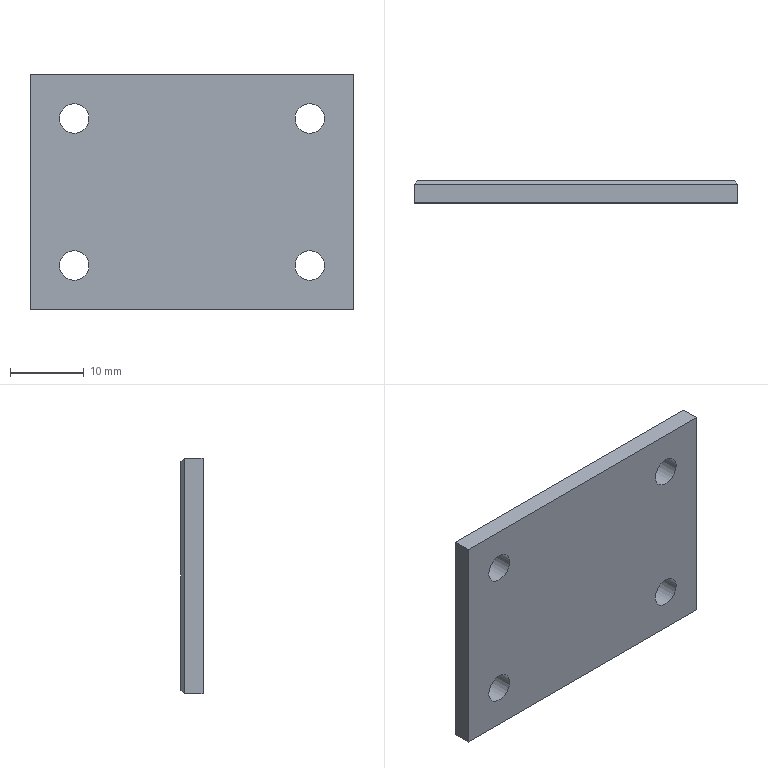Component | NX | END_CAP | 1 solid | 14 faces | box 44 x 3 x 32 mm | volume 4054 mm3 | plane 10 | cylinder 4 | commonest cylinder face diameters 4 x4
STEP:
#1=CARTESIAN_POINT('',(0.,0.,0.));
#2=DIRECTION('',(0.,0.,1.));
#3=DIRECTION('',(1.,0.,0.));
#4=AXIS2_PLACEMENT_3D('',#1,#2,#3);
#5=CARTESIAN_POINT('',(412.5,-54.,127.));
#6=VERTEX_POINT('',#5);
#7=CARTESIAN_POINT('',(412.5,-56.5,127.));
#8=VERTEX_POINT('',#7);
#9=CARTESIAN_POINT('',(412.5,-53.5,127.));
#10=DIRECTION('',(0.,-1.,0.));
#11=VECTOR('',#10,1.);
#12=LINE('',#9,#11);
#13=CARTESIAN_POINT('',(412.5,-53.5,127.));
#14=DIRECTION('',(0.,0.,1.));
#15=DIRECTION('',(0.,-1.,0.));
#16=AXIS2_PLACEMENT_3D('',#13,#14,#15);
#17=PLANE('',#16);
#18=CARTESIAN_POINT('',(0.,0.));
#19=DIRECTION('',(1.,0.));
#20=VECTOR('',#19,1.);
#21=LINE('',#18,#20);
#22=(GEOMETRIC_REPRESENTATION_CONTEXT(2)PARAMETRIC_REPRESENTATION_CONTEXT()REPRESENTATION_CONTEXT('',''));
#23=DEFINITIONAL_REPRESENTATION('',(#21),#22);
#24=PCURVE('',#17,#23);
#25=CARTESIAN_POINT('',(412.5,-53.5,95.));
#26=DIRECTION('',(1.,0.,0.));
#27=DIRECTION('',(0.,-1.,0.));
#28=AXIS2_PLACEMENT_3D('',#25,#26,#27);
#29=PLANE('',#28);
#30=CARTESIAN_POINT('',(0.,-32.));
#31=DIRECTION('',(1.,0.));
#32=VECTOR('',#31,1.);
#33=LINE('',#30,#32);
#34=(GEOMETRIC_REPRESENTATION_CONTEXT(2)PARAMETRIC_REPRESENTATION_CONTEXT()REPRESENTATION_CONTEXT('',''));
#35=DEFINITIONAL_REPRESENTATION('',(#33),#34);
#36=PCURVE('',#29,#35);
#37=SURFACE_CURVE('',#12,(#24,#36),.PCURVE_S1.);
#38=EDGE_CURVE('',#6,#8,#37,.T.);
#39=ORIENTED_EDGE('',*,*,#38,.F.);
#40=CARTESIAN_POINT('',(368.5,-54.,127.));
#41=VERTEX_POINT('',#40);
#42=CARTESIAN_POINT('',(412.5,-54.,127.));
#43=DIRECTION('',(-1.,0.,0.));
#44=VECTOR('',#43,1.);
#45=LINE('',#42,#44);
#46=CARTESIAN_POINT('',(0.5,0.));
#47=DIRECTION('',(0.,-1.));
#48=VECTOR('',#47,1.);
#49=LINE('',#46,#48);
#50=(GEOMETRIC_REPRESENTATION_CONTEXT(2)PARAMETRIC_REPRESENTATION_CONTEXT()REPRESENTATION_CONTEXT('',''));
#51=DEFINITIONAL_REPRESENTATION('',(#49),#50);
#52=PCURVE('',#17,#51);
#53=CARTESIAN_POINT('',(412.5,-54.,127.));
#54=DIRECTION('',(0.,-0.7071,-0.7071));
#55=DIRECTION('',(-1.,0.,0.));
#56=AXIS2_PLACEMENT_3D('',#53,#54,#55);
#57=PLANE('',#56);
#58=CARTESIAN_POINT('',(0.,0.));
#59=DIRECTION('',(1.,0.));
#60=VECTOR('',#59,1.);
#61=LINE('',#58,#60);
#62=(GEOMETRIC_REPRESENTATION_CONTEXT(2)PARAMETRIC_REPRESENTATION_CONTEXT()REPRESENTATION_CONTEXT('',''));
#63=DEFINITIONAL_REPRESENTATION('',(#61),#62);
#64=PCURVE('',#57,#63);
#65=SURFACE_CURVE('',#45,(#52,#64),.PCURVE_S1.);
#66=EDGE_CURVE('',#6,#41,#65,.T.);
#67=ORIENTED_EDGE('',*,*,#66,.T.);
#68=CARTESIAN_POINT('',(368.5,-56.5,127.));
#69=VERTEX_POINT('',#68);
#70=CARTESIAN_POINT('',(368.5,-53.5,127.));
#71=DIRECTION('',(0.,-1.,0.));
#72=VECTOR('',#71,1.);
#73=LINE('',#70,#72);
#74=CARTESIAN_POINT('',(0.,-44.));
#75=DIRECTION('',(1.,0.));
#76=VECTOR('',#75,1.);
#77=LINE('',#74,#76);
#78=(GEOMETRIC_REPRESENTATION_CONTEXT(2)PARAMETRIC_REPRESENTATION_CONTEXT()REPRESENTATION_CONTEXT('',''));
#79=DEFINITIONAL_REPRESENTATION('',(#77),#78);
#80=PCURVE('',#17,#79);
#81=CARTESIAN_POINT('',(368.5,-53.5,127.));
#82=DIRECTION('',(-1.,0.,0.));
#83=DIRECTION('',(0.,1.,0.));
#84=AXIS2_PLACEMENT_3D('',#81,#82,#83);
#85=PLANE('',#84);
#86=CARTESIAN_POINT('',(0.,0.));
#87=DIRECTION('',(-1.,0.));
#88=VECTOR('',#87,1.);
#89=LINE('',#86,#88);
#90=(GEOMETRIC_REPRESENTATION_CONTEXT(2)PARAMETRIC_REPRESENTATION_CONTEXT()REPRESENTATION_CONTEXT('',''));
#91=DEFINITIONAL_REPRESENTATION('',(#89),#90);
#92=PCURVE('',#85,#91);
#93=SURFACE_CURVE('',#73,(#80,#92),.PCURVE_S1.);
#94=EDGE_CURVE('',#41,#69,#93,.T.);
#95=ORIENTED_EDGE('',*,*,#94,.T.);
#96=CARTESIAN_POINT('',(412.5,-56.5,127.));
#97=DIRECTION('',(-1.,0.,0.));
#98=VECTOR('',#97,1.);
#99=LINE('',#96,#98);
#100=CARTESIAN_POINT('',(3.,0.));
#101=DIRECTION('',(0.,-1.));
#102=VECTOR('',#101,1.);
#103=LINE('',#100,#102);
#104=(GEOMETRIC_REPRESENTATION_CONTEXT(2)PARAMETRIC_REPRESENTATION_CONTEXT()REPRESENTATION_CONTEXT('',''));
#105=DEFINITIONAL_REPRESENTATION('',(#103),#104);
#106=PCURVE('',#17,#105);
#107=CARTESIAN_POINT('',(406.5,-56.5,101.));
#108=DIRECTION('',(0.,1.,0.));
#109=DIRECTION('',(1.,0.,0.));
#110=AXIS2_PLACEMENT_3D('',#107,#108,#109);
#111=PLANE('',#110);
#112=CARTESIAN_POINT('',(6.,-26.));
#113=DIRECTION('',(-1.,0.));
#114=VECTOR('',#113,1.);
#115=LINE('',#112,#114);
#116=(GEOMETRIC_REPRESENTATION_CONTEXT(2)PARAMETRIC_REPRESENTATION_CONTEXT()REPRESENTATION_CONTEXT('',''));
#117=DEFINITIONAL_REPRESENTATION('',(#115),#116);
#118=PCURVE('',#111,#117);
#119=SURFACE_CURVE('',#99,(#106,#118),.PCURVE_S1.);
#120=EDGE_CURVE('',#8,#69,#119,.T.);
#121=ORIENTED_EDGE('',*,*,#120,.F.);
#122=EDGE_LOOP('',(#39,#67,#95,#121));
#123=FACE_BOUND('',#122,.T.);
#124=ADVANCED_FACE('',(#123),#17,.T.);
#125=ORIENTED_EDGE('',*,*,#94,.F.);
#126=CARTESIAN_POINT('',(368.5,-54.,95.));
#127=VERTEX_POINT('',#126);
#128=CARTESIAN_POINT('',(368.5,-54.,127.));
#129=DIRECTION('',(0.,0.,-1.));
#130=VECTOR('',#129,1.);
#131=LINE('',#128,#130);
#132=CARTESIAN_POINT('',(-0.5,0.));
#133=DIRECTION('',(0.,1.));
#134=VECTOR('',#133,1.);
#135=LINE('',#132,#134);
#136=(GEOMETRIC_REPRESENTATION_CONTEXT(2)PARAMETRIC_REPRESENTATION_CONTEXT()REPRESENTATION_CONTEXT('',''));
#137=DEFINITIONAL_REPRESENTATION('',(#135),#136);
#138=PCURVE('',#85,#137);
#139=CARTESIAN_POINT('',(368.5,-54.,127.));
#140=DIRECTION('',(0.7071,-0.7071,0.));
#141=DIRECTION('',(0.,0.,-1.));
#142=AXIS2_PLACEMENT_3D('',#139,#140,#141);
#143=PLANE('',#142);
#144=CARTESIAN_POINT('',(0.,0.));
#145=DIRECTION('',(1.,0.));
#146=VECTOR('',#145,1.);
#147=LINE('',#144,#146);
#148=(GEOMETRIC_REPRESENTATION_CONTEXT(2)PARAMETRIC_REPRESENTATION_CONTEXT()REPRESENTATION_CONTEXT('',''));
#149=DEFINITIONAL_REPRESENTATION('',(#147),#148);
#150=PCURVE('',#143,#149);
#151=SURFACE_CURVE('',#131,(#138,#150),.PCURVE_S1.);
#152=EDGE_CURVE('',#41,#127,#151,.T.);
#153=ORIENTED_EDGE('',*,*,#152,.T.);
#154=CARTESIAN_POINT('',(368.5,-56.5,95.));
#155=VERTEX_POINT('',#154);
#156=CARTESIAN_POINT('',(368.5,-53.5,95.));
#157=DIRECTION('',(0.,-1.,0.));
#158=VECTOR('',#157,1.);
#159=LINE('',#156,#158);
#160=CARTESIAN_POINT('',(0.,32.));
#161=DIRECTION('',(-1.,0.));
#162=VECTOR('',#161,1.);
#163=LINE('',#160,#162);
#164=(GEOMETRIC_REPRESENTATION_CONTEXT(2)PARAMETRIC_REPRESENTATION_CONTEXT()REPRESENTATION_CONTEXT('',''));
#165=DEFINITIONAL_REPRESENTATION('',(#163),#164);
#166=PCURVE('',#85,#165);
#167=CARTESIAN_POINT('',(368.5,-53.5,95.));
#168=DIRECTION('',(0.,0.,-1.));
#169=DIRECTION('',(0.,1.,0.));
#170=AXIS2_PLACEMENT_3D('',#167,#168,#169);
#171=PLANE('',#170);
#172=CARTESIAN_POINT('',(0.,0.));
#173=DIRECTION('',(-1.,0.));
#174=VECTOR('',#173,1.);
#175=LINE('',#172,#174);
#176=(GEOMETRIC_REPRESENTATION_CONTEXT(2)PARAMETRIC_REPRESENTATION_CONTEXT()REPRESENTATION_CONTEXT('',''));
#177=DEFINITIONAL_REPRESENTATION('',(#175),#176);
#178=PCURVE('',#171,#177);
#179=SURFACE_CURVE('',#159,(#166,#178),.PCURVE_S1.);
#180=EDGE_CURVE('',#127,#155,#179,.T.);
#181=ORIENTED_EDGE('',*,*,#180,.T.);
#182=CARTESIAN_POINT('',(368.5,-56.5,127.));
#183=DIRECTION('',(0.,0.,-1.));
#184=VECTOR('',#183,1.);
#185=LINE('',#182,#184);
#186=CARTESIAN_POINT('',(-3.,0.));
#187=DIRECTION('',(0.,1.));
#188=VECTOR('',#187,1.);
#189=LINE('',#186,#188);
#190=(GEOMETRIC_REPRESENTATION_CONTEXT(2)PARAMETRIC_REPRESENTATION_CONTEXT()REPRESENTATION_CONTEXT('',''));
#191=DEFINITIONAL_REPRESENTATION('',(#189),#190);
#192=PCURVE('',#85,#191);
#193=CARTESIAN_POINT('',(-38.,-26.));
#194=DIRECTION('',(0.,1.));
#195=VECTOR('',#194,1.);
#196=LINE('',#193,#195);
#197=(GEOMETRIC_REPRESENTATION_CONTEXT(2)PARAMETRIC_REPRESENTATION_CONTEXT()REPRESENTATION_CONTEXT('',''));
#198=DEFINITIONAL_REPRESENTATION('',(#196),#197);
#199=PCURVE('',#111,#198);
#200=SURFACE_CURVE('',#185,(#192,#199),.PCURVE_S1.);
#201=EDGE_CURVE('',#69,#155,#200,.T.);
#202=ORIENTED_EDGE('',*,*,#201,.F.);
#203=EDGE_LOOP('',(#125,#153,#181,#202));
#204=FACE_BOUND('',#203,.T.);
#205=ADVANCED_FACE('',(#204),#85,.T.);
#206=ORIENTED_EDGE('',*,*,#180,.F.);
#207=CARTESIAN_POINT('',(412.5,-54.,95.));
#208=VERTEX_POINT('',#207);
#209=CARTESIAN_POINT('',(368.5,-54.,95.));
#210=DIRECTION('',(1.,0.,0.));
#211=VECTOR('',#210,1.);
#212=LINE('',#209,#211);
#213=CARTESIAN_POINT('',(-0.5,0.));
#214=DIRECTION('',(0.,1.));
#215=VECTOR('',#214,1.);
#216=LINE('',#213,#215);
#217=(GEOMETRIC_REPRESENTATION_CONTEXT(2)PARAMETRIC_REPRESENTATION_CONTEXT()REPRESENTATION_CONTEXT('',''));
#218=DEFINITIONAL_REPRESENTATION('',(#216),#217);
#219=PCURVE('',#171,#218);
#220=CARTESIAN_POINT('',(368.5,-54.,95.));
#221=DIRECTION('',(0.,-0.7071,0.7071));
#222=DIRECTION('',(1.,0.,0.));
#223=AXIS2_PLACEMENT_3D('',#220,#221,#222);
#224=PLANE('',#223);
#225=CARTESIAN_POINT('',(0.,0.));
#226=DIRECTION('',(1.,0.));
#227=VECTOR('',#226,1.);
#228=LINE('',#225,#227);
#229=(GEOMETRIC_REPRESENTATION_CONTEXT(2)PARAMETRIC_REPRESENTATION_CONTEXT()REPRESENTATION_CONTEXT('',''));
#230=DEFINITIONAL_REPRESENTATION('',(#228),#229);
#231=PCURVE('',#224,#230);
#232=SURFACE_CURVE('',#212,(#219,#231),.PCURVE_S1.);
#233=EDGE_CURVE('',#127,#208,#232,.T.);
#234=ORIENTED_EDGE('',*,*,#233,.T.);
#235=CARTESIAN_POINT('',(412.5,-56.5,95.));
#236=VERTEX_POINT('',#235);
#237=CARTESIAN_POINT('',(412.5,-53.5,95.));
#238=DIRECTION('',(0.,-1.,0.));
#239=VECTOR('',#238,1.);
#240=LINE('',#237,#239);
#241=CARTESIAN_POINT('',(0.,44.));
#242=DIRECTION('',(-1.,0.));
#243=VECTOR('',#242,1.);
#244=LINE('',#241,#243);
#245=(GEOMETRIC_REPRESENTATION_CONTEXT(2)PARAMETRIC_REPRESENTATION_CONTEXT()REPRESENTATION_CONTEXT('',''));
#246=DEFINITIONAL_REPRESENTATION('',(#244),#245);
#247=PCURVE('',#171,#246);
#248=CARTESIAN_POINT('',(0.,0.));
#249=DIRECTION('',(1.,0.));
#250=VECTOR('',#249,1.);
#251=LINE('',#248,#250);
#252=(GEOMETRIC_REPRESENTATION_CONTEXT(2)PARAMETRIC_REPRESENTATION_CONTEXT()REPRESENTATION_CONTEXT('',''));
#253=DEFINITIONAL_REPRESENTATION('',(#251),#252);
#254=PCURVE('',#29,#253);
#255=SURFACE_CURVE('',#240,(#247,#254),.PCURVE_S1.);
#256=EDGE_CURVE('',#208,#236,#255,.T.);
#257=ORIENTED_EDGE('',*,*,#256,.T.);
#258=CARTESIAN_POINT('',(368.5,-56.5,95.));
#259=DIRECTION('',(1.,0.,0.));
#260=VECTOR('',#259,1.);
#261=LINE('',#258,#260);
#262=CARTESIAN_POINT('',(-3.,0.));
#263=DIRECTION('',(0.,1.));
#264=VECTOR('',#263,1.);
#265=LINE('',#262,#264);
#266=(GEOMETRIC_REPRESENTATION_CONTEXT(2)PARAMETRIC_REPRESENTATION_CONTEXT()REPRESENTATION_CONTEXT('',''));
#267=DEFINITIONAL_REPRESENTATION('',(#265),#266);
#268=PCURVE('',#171,#267);
#269=CARTESIAN_POINT('',(-38.,6.));
#270=DIRECTION('',(1.,0.));
#271=VECTOR('',#270,1.);
#272=LINE('',#269,#271);
#273=(GEOMETRIC_REPRESENTATION_CONTEXT(2)PARAMETRIC_REPRESENTATION_CONTEXT()REPRESENTATION_CONTEXT('',''));
#274=DEFINITIONAL_REPRESENTATION('',(#272),#273);
#275=PCURVE('',#111,#274);
#276=SURFACE_CURVE('',#261,(#268,#275),.PCURVE_S1.);
#277=EDGE_CURVE('',#155,#236,#276,.T.);
#278=ORIENTED_EDGE('',*,*,#277,.F.);
#279=EDGE_LOOP('',(#206,#234,#257,#278));
#280=FACE_BOUND('',#279,.T.);
#281=ADVANCED_FACE('',(#280),#171,.T.);
#282=CARTESIAN_POINT('',(376.5,-53.5,121.));
#283=VERTEX_POINT('',#282);
#284=CARTESIAN_POINT('',(374.5,-53.5,121.));
#285=DIRECTION('',(0.,1.,0.));
#286=DIRECTION('',(1.,0.,0.));
#287=AXIS2_PLACEMENT_3D('',#284,#285,#286);
#288=CIRCLE('',#287,2.);
#289=CARTESIAN_POINT('',(374.5,-53.5,121.));
#290=DIRECTION('',(0.,-1.,0.));
#291=DIRECTION('',(-1.,0.,0.));
#292=AXIS2_PLACEMENT_3D('',#289,#290,#291);
#293=CYLINDRICAL_SURFACE('',#292,2.);
#294=CARTESIAN_POINT('',(9.425,0.));
#295=DIRECTION('',(-1.,0.));
#296=VECTOR('',#295,1.);
#297=LINE('',#294,#296);
#298=(GEOMETRIC_REPRESENTATION_CONTEXT(2)PARAMETRIC_REPRESENTATION_CONTEXT()REPRESENTATION_CONTEXT('',''));
#299=DEFINITIONAL_REPRESENTATION('',(#297),#298);
#300=PCURVE('',#293,#299);
#301=CARTESIAN_POINT('',(406.5,-53.5,101.));
#302=DIRECTION('',(0.,1.,0.));
#303=DIRECTION('',(1.,0.,0.));
#304=AXIS2_PLACEMENT_3D('',#301,#302,#303);
#305=PLANE('',#304);
#306=CARTESIAN_POINT('',(-32.,-20.));
#307=DIRECTION('',(1.,0.));
#308=AXIS2_PLACEMENT_2D('',#306,#307);
#309=CIRCLE('',#308,2.);
#310=(GEOMETRIC_REPRESENTATION_CONTEXT(2)PARAMETRIC_REPRESENTATION_CONTEXT()REPRESENTATION_CONTEXT('',''));
#311=DEFINITIONAL_REPRESENTATION('',(#309),#310);
#312=PCURVE('',#305,#311);
#313=SURFACE_CURVE('',#288,(#300,#312),.PCURVE_S1.);
#314=EDGE_CURVE('',#283,#283,#313,.T.);
#315=ORIENTED_EDGE('',*,*,#314,.F.);
#316=CARTESIAN_POINT('',(376.5,-56.5,121.));
#317=VERTEX_POINT('',#316);
#318=CARTESIAN_POINT('',(376.5,-53.5,121.));
#319=CARTESIAN_POINT('',(376.5,-56.5,121.));
#320=B_SPLINE_CURVE_WITH_KNOTS('',1,(#318,#319),.UNSPECIFIED.,.F.,.F.,(2,2),(0.,3.),.PIECEWISE_BEZIER_KNOTS.);
#321=CARTESIAN_POINT('',(9.425,0.));
#322=DIRECTION('',(0.,1.));
#323=VECTOR('',#322,1.);
#324=LINE('',#321,#323);
#325=(GEOMETRIC_REPRESENTATION_CONTEXT(2)PARAMETRIC_REPRESENTATION_CONTEXT()REPRESENTATION_CONTEXT('',''));
#326=DEFINITIONAL_REPRESENTATION('',(#324),#325);
#327=PCURVE('',#293,#326);
#328=CARTESIAN_POINT('',(3.142,0.));
#329=DIRECTION('',(0.,1.));
#330=VECTOR('',#329,1.);
#331=LINE('',#328,#330);
#332=(GEOMETRIC_REPRESENTATION_CONTEXT(2)PARAMETRIC_REPRESENTATION_CONTEXT()REPRESENTATION_CONTEXT('',''));
#333=DEFINITIONAL_REPRESENTATION('',(#331),#332);
#334=PCURVE('',#293,#333);
#335=SEAM_CURVE('',#320,(#327,#334),.PCURVE_S1.);
#336=EDGE_CURVE('',#283,#317,#335,.T.);
#337=ORIENTED_EDGE('',*,*,#336,.T.);
#338=CARTESIAN_POINT('',(374.5,-56.5,121.));
#339=DIRECTION('',(0.,1.,0.));
#340=DIRECTION('',(1.,0.,0.));
#341=AXIS2_PLACEMENT_3D('',#338,#339,#340);
#342=CIRCLE('',#341,2.);
#343=CARTESIAN_POINT('',(9.425,3.));
#344=DIRECTION('',(-1.,0.));
#345=VECTOR('',#344,1.);
#346=LINE('',#343,#345);
#347=(GEOMETRIC_REPRESENTATION_CONTEXT(2)PARAMETRIC_REPRESENTATION_CONTEXT()REPRESENTATION_CONTEXT('',''));
#348=DEFINITIONAL_REPRESENTATION('',(#346),#347);
#349=PCURVE('',#293,#348);
#350=CARTESIAN_POINT('',(-32.,-20.));
#351=DIRECTION('',(1.,0.));
#352=AXIS2_PLACEMENT_2D('',#350,#351);
#353=CIRCLE('',#352,2.);
#354=(GEOMETRIC_REPRESENTATION_CONTEXT(2)PARAMETRIC_REPRESENTATION_CONTEXT()REPRESENTATION_CONTEXT('',''));
#355=DEFINITIONAL_REPRESENTATION('',(#353),#354);
#356=PCURVE('',#111,#355);
#357=SURFACE_CURVE('',#342,(#349,#356),.PCURVE_S1.);
#358=EDGE_CURVE('',#317,#317,#357,.T.);
#359=ORIENTED_EDGE('',*,*,#358,.T.);
#360=ORIENTED_EDGE('',*,*,#336,.F.);
#361=EDGE_LOOP('',(#315,#337,#359,#360));
#362=FACE_BOUND('',#361,.F.);
#363=ADVANCED_FACE('',(#362),#293,.F.);
#364=CARTESIAN_POINT('',(376.5,-53.5,101.));
#365=VERTEX_POINT('',#364);
#366=CARTESIAN_POINT('',(374.5,-53.5,101.));
#367=DIRECTION('',(0.,-1.,0.));
#368=DIRECTION('',(1.,0.,0.));
#369=AXIS2_PLACEMENT_3D('',#366,#367,#368);
#370=CIRCLE('',#369,2.);
#371=CARTESIAN_POINT('',(374.5,-53.5,101.));
#372=DIRECTION('',(0.,-1.,0.));
#373=DIRECTION('',(-1.,0.,0.));
#374=AXIS2_PLACEMENT_3D('',#371,#372,#373);
#375=CYLINDRICAL_SURFACE('',#374,2.);
#376=CARTESIAN_POINT('',(3.142,0.));
#377=DIRECTION('',(1.,0.));
#378=VECTOR('',#377,1.);
#379=LINE('',#376,#378);
#380=(GEOMETRIC_REPRESENTATION_CONTEXT(2)PARAMETRIC_REPRESENTATION_CONTEXT()REPRESENTATION_CONTEXT('',''));
#381=DEFINITIONAL_REPRESENTATION('',(#379),#380);
#382=PCURVE('',#375,#381);
#383=CARTESIAN_POINT('',(-30.,0.));
#384=CARTESIAN_POINT('',(-30.,-3.464));
#385=CARTESIAN_POINT('',(-33.,-1.732));
#386=CARTESIAN_POINT('',(-36.,-0.));
#387=CARTESIAN_POINT('',(-33.,1.732));
#388=CARTESIAN_POINT('',(-30.,3.464));
#389=CARTESIAN_POINT('',(-30.,0.));
#390=(BOUNDED_CURVE()B_SPLINE_CURVE(2,(#383,#384,#385,#386,#387,#388,#389),.UNSPECIFIED.,.T.,.F.)B_SPLINE_CURVE_WITH_KNOTS((1,2,2,2,2,1),(-2.094,0.,2.094,4.189,6.283,8.378),.UNSPECIFIED.)CURVE()GEOMETRIC_REPRESENTATION_ITEM()RATIONAL_B_SPLINE_CURVE((1.,0.5,1.,0.5,1.,0.5,1.))REPRESENTATION_ITEM(''));
#391=(GEOMETRIC_REPRESENTATION_CONTEXT(2)PARAMETRIC_REPRESENTATION_CONTEXT()REPRESENTATION_CONTEXT('',''));
#392=DEFINITIONAL_REPRESENTATION('',(#390),#391);
#393=PCURVE('',#305,#392);
#394=SURFACE_CURVE('',#370,(#382,#393),.PCURVE_S1.);
#395=EDGE_CURVE('',#365,#365,#394,.T.);
#396=ORIENTED_EDGE('',*,*,#395,.T.);
#397=CARTESIAN_POINT('',(376.5,-56.5,101.));
#398=VERTEX_POINT('',#397);
#399=CARTESIAN_POINT('',(376.5,-53.5,101.));
#400=CARTESIAN_POINT('',(376.5,-56.5,101.));
#401=B_SPLINE_CURVE_WITH_KNOTS('',1,(#399,#400),.UNSPECIFIED.,.F.,.F.,(2,2),(0.,3.),.PIECEWISE_BEZIER_KNOTS.);
#402=CARTESIAN_POINT('',(9.425,0.));
#403=DIRECTION('',(0.,1.));
#404=VECTOR('',#403,1.);
#405=LINE('',#402,#404);
#406=(GEOMETRIC_REPRESENTATION_CONTEXT(2)PARAMETRIC_REPRESENTATION_CONTEXT()REPRESENTATION_CONTEXT('',''));
#407=DEFINITIONAL_REPRESENTATION('',(#405),#406);
#408=PCURVE('',#375,#407);
#409=CARTESIAN_POINT('',(3.142,0.));
#410=DIRECTION('',(0.,1.));
#411=VECTOR('',#410,1.);
#412=LINE('',#409,#411);
#413=(GEOMETRIC_REPRESENTATION_CONTEXT(2)PARAMETRIC_REPRESENTATION_CONTEXT()REPRESENTATION_CONTEXT('',''));
#414=DEFINITIONAL_REPRESENTATION('',(#412),#413);
#415=PCURVE('',#375,#414);
#416=SEAM_CURVE('',#401,(#408,#415),.PCURVE_S1.);
#417=EDGE_CURVE('',#365,#398,#416,.T.);
#418=ORIENTED_EDGE('',*,*,#417,.T.);
#419=CARTESIAN_POINT('',(374.5,-56.5,101.));
#420=DIRECTION('',(0.,-1.,0.));
#421=DIRECTION('',(1.,0.,0.));
#422=AXIS2_PLACEMENT_3D('',#419,#420,#421);
#423=CIRCLE('',#422,2.);
#424=CARTESIAN_POINT('',(3.142,3.));
#425=DIRECTION('',(1.,0.));
#426=VECTOR('',#425,1.);
#427=LINE('',#424,#426);
#428=(GEOMETRIC_REPRESENTATION_CONTEXT(2)PARAMETRIC_REPRESENTATION_CONTEXT()REPRESENTATION_CONTEXT('',''));
#429=DEFINITIONAL_REPRESENTATION('',(#427),#428);
#430=PCURVE('',#375,#429);
#431=CARTESIAN_POINT('',(-30.,0.));
#432=CARTESIAN_POINT('',(-30.,-3.464));
#433=CARTESIAN_POINT('',(-33.,-1.732));
#434=CARTESIAN_POINT('',(-36.,-0.));
#435=CARTESIAN_POINT('',(-33.,1.732));
#436=CARTESIAN_POINT('',(-30.,3.464));
#437=CARTESIAN_POINT('',(-30.,0.));
#438=(BOUNDED_CURVE()B_SPLINE_CURVE(2,(#431,#432,#433,#434,#435,#436,#437),.UNSPECIFIED.,.T.,.F.)B_SPLINE_CURVE_WITH_KNOTS((1,2,2,2,2,1),(-2.094,0.,2.094,4.189,6.283,8.378),.UNSPECIFIED.)CURVE()GEOMETRIC_REPRESENTATION_ITEM()RATIONAL_B_SPLINE_CURVE((1.,0.5,1.,0.5,1.,0.5,1.))REPRESENTATION_ITEM(''));
#439=(GEOMETRIC_REPRESENTATION_CONTEXT(2)PARAMETRIC_REPRESENTATION_CONTEXT()REPRESENTATION_CONTEXT('',''));
#440=DEFINITIONAL_REPRESENTATION('',(#438),#439);
#441=PCURVE('',#111,#440);
#442=SURFACE_CURVE('',#423,(#430,#441),.PCURVE_S1.);
#443=EDGE_CURVE('',#398,#398,#442,.T.);
#444=ORIENTED_EDGE('',*,*,#443,.F.);
#445=ORIENTED_EDGE('',*,*,#417,.F.);
#446=EDGE_LOOP('',(#396,#418,#444,#445));
#447=FACE_BOUND('',#446,.F.);
#448=ADVANCED_FACE('',(#447),#375,.F.);
#449=CARTESIAN_POINT('',(404.5,-53.5,101.));
#450=VERTEX_POINT('',#449);
#451=CARTESIAN_POINT('',(406.5,-53.5,101.));
#452=DIRECTION('',(0.,1.,0.));
#453=DIRECTION('',(-1.,0.,0.));
#454=AXIS2_PLACEMENT_3D('',#451,#452,#453);
#455=CIRCLE('',#454,2.);
#456=CARTESIAN_POINT('',(406.5,-53.5,101.));
#457=DIRECTION('',(0.,-1.,0.));
#458=DIRECTION('',(-1.,0.,0.));
#459=AXIS2_PLACEMENT_3D('',#456,#457,#458);
#460=CYLINDRICAL_SURFACE('',#459,2.);
#461=CARTESIAN_POINT('',(6.283,0.));
#462=DIRECTION('',(-1.,0.));
#463=VECTOR('',#462,1.);
#464=LINE('',#461,#463);
#465=(GEOMETRIC_REPRESENTATION_CONTEXT(2)PARAMETRIC_REPRESENTATION_CONTEXT()REPRESENTATION_CONTEXT('',''));
#466=DEFINITIONAL_REPRESENTATION('',(#464),#465);
#467=PCURVE('',#460,#466);
#468=CARTESIAN_POINT('',(0.,0.));
#469=DIRECTION('',(-1.,0.));
#470=AXIS2_PLACEMENT_2D('',#468,#469);
#471=CIRCLE('',#470,2.);
#472=(GEOMETRIC_REPRESENTATION_CONTEXT(2)PARAMETRIC_REPRESENTATION_CONTEXT()REPRESENTATION_CONTEXT('',''));
#473=DEFINITIONAL_REPRESENTATION('',(#471),#472);
#474=PCURVE('',#305,#473);
#475=SURFACE_CURVE('',#455,(#467,#474),.PCURVE_S1.);
#476=EDGE_CURVE('',#450,#450,#475,.T.);
#477=ORIENTED_EDGE('',*,*,#476,.F.);
#478=CARTESIAN_POINT('',(404.5,-56.5,101.));
#479=VERTEX_POINT('',#478);
#480=CARTESIAN_POINT('',(404.5,-53.5,101.));
#481=CARTESIAN_POINT('',(404.5,-56.5,101.));
#482=B_SPLINE_CURVE_WITH_KNOTS('',1,(#480,#481),.UNSPECIFIED.,.F.,.F.,(2,2),(0.,3.),.PIECEWISE_BEZIER_KNOTS.);
#483=CARTESIAN_POINT('',(6.283,0.));
#484=DIRECTION('',(0.,1.));
#485=VECTOR('',#484,1.);
#486=LINE('',#483,#485);
#487=(GEOMETRIC_REPRESENTATION_CONTEXT(2)PARAMETRIC_REPRESENTATION_CONTEXT()REPRESENTATION_CONTEXT('',''));
#488=DEFINITIONAL_REPRESENTATION('',(#486),#487);
#489=PCURVE('',#460,#488);
#490=CARTESIAN_POINT('',(0.,0.));
#491=DIRECTION('',(0.,1.));
#492=VECTOR('',#491,1.);
#493=LINE('',#490,#492);
#494=(GEOMETRIC_REPRESENTATION_CONTEXT(2)PARAMETRIC_REPRESENTATION_CONTEXT()REPRESENTATION_CONTEXT('',''));
#495=DEFINITIONAL_REPRESENTATION('',(#493),#494);
#496=PCURVE('',#460,#495);
#497=SEAM_CURVE('',#482,(#489,#496),.PCURVE_S1.);
#498=EDGE_CURVE('',#450,#479,#497,.T.);
#499=ORIENTED_EDGE('',*,*,#498,.T.);
#500=CARTESIAN_POINT('',(406.5,-56.5,101.));
#501=DIRECTION('',(0.,1.,0.));
#502=DIRECTION('',(-1.,0.,0.));
#503=AXIS2_PLACEMENT_3D('',#500,#501,#502);
#504=CIRCLE('',#503,2.);
#505=CARTESIAN_POINT('',(6.283,3.));
#506=DIRECTION('',(-1.,0.));
#507=VECTOR('',#506,1.);
#508=LINE('',#505,#507);
#509=(GEOMETRIC_REPRESENTATION_CONTEXT(2)PARAMETRIC_REPRESENTATION_CONTEXT()REPRESENTATION_CONTEXT('',''));
#510=DEFINITIONAL_REPRESENTATION('',(#508),#509);
#511=PCURVE('',#460,#510);
#512=CARTESIAN_POINT('',(0.,0.));
#513=DIRECTION('',(-1.,0.));
#514=AXIS2_PLACEMENT_2D('',#512,#513);
#515=CIRCLE('',#514,2.);
#516=(GEOMETRIC_REPRESENTATION_CONTEXT(2)PARAMETRIC_REPRESENTATION_CONTEXT()REPRESENTATION_CONTEXT('',''));
#517=DEFINITIONAL_REPRESENTATION('',(#515),#516);
#518=PCURVE('',#111,#517);
#519=SURFACE_CURVE('',#504,(#511,#518),.PCURVE_S1.);
#520=EDGE_CURVE('',#479,#479,#519,.T.);
#521=ORIENTED_EDGE('',*,*,#520,.T.);
#522=ORIENTED_EDGE('',*,*,#498,.F.);
#523=EDGE_LOOP('',(#477,#499,#521,#522));
#524=FACE_BOUND('',#523,.F.);
#525=ADVANCED_FACE('',(#524),#460,.F.);
#526=ORIENTED_EDGE('',*,*,#256,.F.);
#527=CARTESIAN_POINT('',(412.5,-54.,95.));
#528=DIRECTION('',(0.,0.,1.));
#529=VECTOR('',#528,1.);
#530=LINE('',#527,#529);
#531=CARTESIAN_POINT('',(0.5,0.));
#532=DIRECTION('',(0.,-1.));
#533=VECTOR('',#532,1.);
#534=LINE('',#531,#533);
#535=(GEOMETRIC_REPRESENTATION_CONTEXT(2)PARAMETRIC_REPRESENTATION_CONTEXT()REPRESENTATION_CONTEXT('',''));
#536=DEFINITIONAL_REPRESENTATION('',(#534),#535);
#537=PCURVE('',#29,#536);
#538=CARTESIAN_POINT('',(412.5,-54.,95.));
#539=DIRECTION('',(-0.7071,-0.7071,0.));
#540=DIRECTION('',(0.,0.,1.));
#541=AXIS2_PLACEMENT_3D('',#538,#539,#540);
#542=PLANE('',#541);
#543=CARTESIAN_POINT('',(0.,0.));
#544=DIRECTION('',(1.,0.));
#545=VECTOR('',#544,1.);
#546=LINE('',#543,#545);
#547=(GEOMETRIC_REPRESENTATION_CONTEXT(2)PARAMETRIC_REPRESENTATION_CONTEXT()REPRESENTATION_CONTEXT('',''));
#548=DEFINITIONAL_REPRESENTATION('',(#546),#547);
#549=PCURVE('',#542,#548);
#550=SURFACE_CURVE('',#530,(#537,#549),.PCURVE_S1.);
#551=EDGE_CURVE('',#208,#6,#550,.T.);
#552=ORIENTED_EDGE('',*,*,#551,.T.);
#553=ORIENTED_EDGE('',*,*,#38,.T.);
#554=CARTESIAN_POINT('',(412.5,-56.5,95.));
#555=DIRECTION('',(0.,0.,1.));
#556=VECTOR('',#555,1.);
#557=LINE('',#554,#556);
#558=CARTESIAN_POINT('',(3.,0.));
#559=DIRECTION('',(0.,-1.));
#560=VECTOR('',#559,1.);
#561=LINE('',#558,#560);
#562=(GEOMETRIC_REPRESENTATION_CONTEXT(2)PARAMETRIC_REPRESENTATION_CONTEXT()REPRESENTATION_CONTEXT('',''));
#563=DEFINITIONAL_REPRESENTATION('',(#561),#562);
#564=PCURVE('',#29,#563);
#565=CARTESIAN_POINT('',(6.,6.));
#566=DIRECTION('',(0.,-1.));
#567=VECTOR('',#566,1.);
#568=LINE('',#565,#567);
#569=(GEOMETRIC_REPRESENTATION_CONTEXT(2)PARAMETRIC_REPRESENTATION_CONTEXT()REPRESENTATION_CONTEXT('',''));
#570=DEFINITIONAL_REPRESENTATION('',(#568),#569);
#571=PCURVE('',#111,#570);
#572=SURFACE_CURVE('',#557,(#564,#571),.PCURVE_S1.);
#573=EDGE_CURVE('',#236,#8,#572,.T.);
#574=ORIENTED_EDGE('',*,*,#573,.F.);
#575=EDGE_LOOP('',(#526,#552,#553,#574));
#576=FACE_BOUND('',#575,.T.);
#577=ADVANCED_FACE('',(#576),#29,.T.);
#578=CARTESIAN_POINT('',(404.5,-53.5,121.));
#579=VERTEX_POINT('',#578);
#580=CARTESIAN_POINT('',(406.5,-53.5,121.));
#581=DIRECTION('',(0.,-1.,0.));
#582=DIRECTION('',(-1.,0.,0.));
#583=AXIS2_PLACEMENT_3D('',#580,#581,#582);
#584=CIRCLE('',#583,2.);
#585=CARTESIAN_POINT('',(406.5,-53.5,121.));
#586=DIRECTION('',(0.,-1.,0.));
#587=DIRECTION('',(-1.,0.,0.));
#588=AXIS2_PLACEMENT_3D('',#585,#586,#587);
#589=CYLINDRICAL_SURFACE('',#588,2.);
#590=CARTESIAN_POINT('',(0.,0.));
#591=DIRECTION('',(1.,0.));
#592=VECTOR('',#591,1.);
#593=LINE('',#590,#592);
#594=(GEOMETRIC_REPRESENTATION_CONTEXT(2)PARAMETRIC_REPRESENTATION_CONTEXT()REPRESENTATION_CONTEXT('',''));
#595=DEFINITIONAL_REPRESENTATION('',(#593),#594);
#596=PCURVE('',#589,#595);
#597=CARTESIAN_POINT('',(-2.,-20.));
#598=CARTESIAN_POINT('',(-2.,-16.536));
#599=CARTESIAN_POINT('',(1.,-18.268));
#600=CARTESIAN_POINT('',(4.,-20.));
#601=CARTESIAN_POINT('',(1.,-21.732));
#602=CARTESIAN_POINT('',(-2.,-23.464));
#603=CARTESIAN_POINT('',(-2.,-20.));
#604=(BOUNDED_CURVE()B_SPLINE_CURVE(2,(#597,#598,#599,#600,#601,#602,#603),.UNSPECIFIED.,.T.,.F.)B_SPLINE_CURVE_WITH_KNOTS((1,2,2,2,2,1),(-2.094,0.,2.094,4.189,6.283,8.378),.UNSPECIFIED.)CURVE()GEOMETRIC_REPRESENTATION_ITEM()RATIONAL_B_SPLINE_CURVE((1.,0.5,1.,0.5,1.,0.5,1.))REPRESENTATION_ITEM(''));
#605=(GEOMETRIC_REPRESENTATION_CONTEXT(2)PARAMETRIC_REPRESENTATION_CONTEXT()REPRESENTATION_CONTEXT('',''));
#606=DEFINITIONAL_REPRESENTATION('',(#604),#605);
#607=PCURVE('',#305,#606);
#608=SURFACE_CURVE('',#584,(#596,#607),.PCURVE_S1.);
#609=EDGE_CURVE('',#579,#579,#608,.T.);
#610=ORIENTED_EDGE('',*,*,#609,.T.);
#611=CARTESIAN_POINT('',(404.5,-56.5,121.));
#612=VERTEX_POINT('',#611);
#613=CARTESIAN_POINT('',(404.5,-53.5,121.));
#614=CARTESIAN_POINT('',(404.5,-56.5,121.));
#615=B_SPLINE_CURVE_WITH_KNOTS('',1,(#613,#614),.UNSPECIFIED.,.F.,.F.,(2,2),(0.,3.),.PIECEWISE_BEZIER_KNOTS.);
#616=CARTESIAN_POINT('',(6.283,0.));
#617=DIRECTION('',(0.,1.));
#618=VECTOR('',#617,1.);
#619=LINE('',#616,#618);
#620=(GEOMETRIC_REPRESENTATION_CONTEXT(2)PARAMETRIC_REPRESENTATION_CONTEXT()REPRESENTATION_CONTEXT('',''));
#621=DEFINITIONAL_REPRESENTATION('',(#619),#620);
#622=PCURVE('',#589,#621);
#623=CARTESIAN_POINT('',(0.,0.));
#624=DIRECTION('',(0.,1.));
#625=VECTOR('',#624,1.);
#626=LINE('',#623,#625);
#627=(GEOMETRIC_REPRESENTATION_CONTEXT(2)PARAMETRIC_REPRESENTATION_CONTEXT()REPRESENTATION_CONTEXT('',''));
#628=DEFINITIONAL_REPRESENTATION('',(#626),#627);
#629=PCURVE('',#589,#628);
#630=SEAM_CURVE('',#615,(#622,#629),.PCURVE_S1.);
#631=EDGE_CURVE('',#579,#612,#630,.T.);
#632=ORIENTED_EDGE('',*,*,#631,.T.);
#633=CARTESIAN_POINT('',(406.5,-56.5,121.));
#634=DIRECTION('',(0.,-1.,0.));
#635=DIRECTION('',(-1.,0.,0.));
#636=AXIS2_PLACEMENT_3D('',#633,#634,#635);
#637=CIRCLE('',#636,2.);
#638=CARTESIAN_POINT('',(0.,3.));
#639=DIRECTION('',(1.,0.));
#640=VECTOR('',#639,1.);
#641=LINE('',#638,#640);
#642=(GEOMETRIC_REPRESENTATION_CONTEXT(2)PARAMETRIC_REPRESENTATION_CONTEXT()REPRESENTATION_CONTEXT('',''));
#643=DEFINITIONAL_REPRESENTATION('',(#641),#642);
#644=PCURVE('',#589,#643);
#645=CARTESIAN_POINT('',(-2.,-20.));
#646=CARTESIAN_POINT('',(-2.,-16.536));
#647=CARTESIAN_POINT('',(1.,-18.268));
#648=CARTESIAN_POINT('',(4.,-20.));
#649=CARTESIAN_POINT('',(1.,-21.732));
#650=CARTESIAN_POINT('',(-2.,-23.464));
#651=CARTESIAN_POINT('',(-2.,-20.));
#652=(BOUNDED_CURVE()B_SPLINE_CURVE(2,(#645,#646,#647,#648,#649,#650,#651),.UNSPECIFIED.,.T.,.F.)B_SPLINE_CURVE_WITH_KNOTS((1,2,2,2,2,1),(-2.094,0.,2.094,4.189,6.283,8.378),.UNSPECIFIED.)CURVE()GEOMETRIC_REPRESENTATION_ITEM()RATIONAL_B_SPLINE_CURVE((1.,0.5,1.,0.5,1.,0.5,1.))REPRESENTATION_ITEM(''));
#653=(GEOMETRIC_REPRESENTATION_CONTEXT(2)PARAMETRIC_REPRESENTATION_CONTEXT()REPRESENTATION_CONTEXT('',''));
#654=DEFINITIONAL_REPRESENTATION('',(#652),#653);
#655=PCURVE('',#111,#654);
#656=SURFACE_CURVE('',#637,(#644,#655),.PCURVE_S1.);
#657=EDGE_CURVE('',#612,#612,#656,.T.);
#658=ORIENTED_EDGE('',*,*,#657,.F.);
#659=ORIENTED_EDGE('',*,*,#631,.F.);
#660=EDGE_LOOP('',(#610,#632,#658,#659));
#661=FACE_BOUND('',#660,.F.);
#662=ADVANCED_FACE('',(#661),#589,.F.);
#663=CARTESIAN_POINT('',(369.,-53.5,126.5));
#664=VERTEX_POINT('',#663);
#665=CARTESIAN_POINT('',(412.,-53.5,126.5));
#666=VERTEX_POINT('',#665);
#667=CARTESIAN_POINT('',(406.5,-53.5,126.5));
#668=DIRECTION('',(1.,0.,0.));
#669=VECTOR('',#668,1.);
#670=LINE('',#667,#669);
#671=CARTESIAN_POINT('',(0.,-25.5));
#672=DIRECTION('',(1.,0.));
#673=VECTOR('',#672,1.);
#674=LINE('',#671,#673);
#675=(GEOMETRIC_REPRESENTATION_CONTEXT(2)PARAMETRIC_REPRESENTATION_CONTEXT()REPRESENTATION_CONTEXT('',''));
#676=DEFINITIONAL_REPRESENTATION('',(#674),#675);
#677=PCURVE('',#305,#676);
#678=CARTESIAN_POINT('',(6.,0.7071));
#679=DIRECTION('',(-1.,0.));
#680=VECTOR('',#679,1.);
#681=LINE('',#678,#680);
#682=(GEOMETRIC_REPRESENTATION_CONTEXT(2)PARAMETRIC_REPRESENTATION_CONTEXT()REPRESENTATION_CONTEXT('',''));
#683=DEFINITIONAL_REPRESENTATION('',(#681),#682);
#684=PCURVE('',#57,#683);
#685=SURFACE_CURVE('',#670,(#677,#684),.PCURVE_S1.);
#686=EDGE_CURVE('',#664,#666,#685,.T.);
#687=ORIENTED_EDGE('',*,*,#686,.T.);
#688=CARTESIAN_POINT('',(412.,-53.5,95.5));
#689=VERTEX_POINT('',#688);
#690=CARTESIAN_POINT('',(412.,-53.5,101.));
#691=DIRECTION('',(0.,0.,-1.));
#692=VECTOR('',#691,1.);
#693=LINE('',#690,#692);
#694=CARTESIAN_POINT('',(5.5,0.));
#695=DIRECTION('',(0.,1.));
#696=VECTOR('',#695,1.);
#697=LINE('',#694,#696);
#698=(GEOMETRIC_REPRESENTATION_CONTEXT(2)PARAMETRIC_REPRESENTATION_CONTEXT()REPRESENTATION_CONTEXT('',''));
#699=DEFINITIONAL_REPRESENTATION('',(#697),#698);
#700=PCURVE('',#305,#699);
#701=CARTESIAN_POINT('',(6.,0.7071));
#702=DIRECTION('',(-1.,0.));
#703=VECTOR('',#702,1.);
#704=LINE('',#701,#703);
#705=(GEOMETRIC_REPRESENTATION_CONTEXT(2)PARAMETRIC_REPRESENTATION_CONTEXT()REPRESENTATION_CONTEXT('',''));
#706=DEFINITIONAL_REPRESENTATION('',(#704),#705);
#707=PCURVE('',#542,#706);
#708=SURFACE_CURVE('',#693,(#700,#707),.PCURVE_S1.);
#709=EDGE_CURVE('',#666,#689,#708,.T.);
#710=ORIENTED_EDGE('',*,*,#709,.T.);
#711=CARTESIAN_POINT('',(369.,-53.5,95.5));
#712=VERTEX_POINT('',#711);
#713=CARTESIAN_POINT('',(406.5,-53.5,95.5));
#714=DIRECTION('',(-1.,0.,0.));
#715=VECTOR('',#714,1.);
#716=LINE('',#713,#715);
#717=CARTESIAN_POINT('',(0.,5.5));
#718=DIRECTION('',(-1.,0.));
#719=VECTOR('',#718,1.);
#720=LINE('',#717,#719);
#721=(GEOMETRIC_REPRESENTATION_CONTEXT(2)PARAMETRIC_REPRESENTATION_CONTEXT()REPRESENTATION_CONTEXT('',''));
#722=DEFINITIONAL_REPRESENTATION('',(#720),#721);
#723=PCURVE('',#305,#722);
#724=CARTESIAN_POINT('',(38.,0.7071));
#725=DIRECTION('',(-1.,0.));
#726=VECTOR('',#725,1.);
#727=LINE('',#724,#726);
#728=(GEOMETRIC_REPRESENTATION_CONTEXT(2)PARAMETRIC_REPRESENTATION_CONTEXT()REPRESENTATION_CONTEXT('',''));
#729=DEFINITIONAL_REPRESENTATION('',(#727),#728);
#730=PCURVE('',#224,#729);
#731=SURFACE_CURVE('',#716,(#723,#730),.PCURVE_S1.);
#732=EDGE_CURVE('',#689,#712,#731,.T.);
#733=ORIENTED_EDGE('',*,*,#732,.T.);
#734=CARTESIAN_POINT('',(369.,-53.5,101.));
#735=DIRECTION('',(0.,0.,1.));
#736=VECTOR('',#735,1.);
#737=LINE('',#734,#736);
#738=CARTESIAN_POINT('',(-37.5,0.));
#739=DIRECTION('',(0.,-1.));
#740=VECTOR('',#739,1.);
#741=LINE('',#738,#740);
#742=(GEOMETRIC_REPRESENTATION_CONTEXT(2)PARAMETRIC_REPRESENTATION_CONTEXT()REPRESENTATION_CONTEXT('',''));
#743=DEFINITIONAL_REPRESENTATION('',(#741),#742);
#744=PCURVE('',#305,#743);
#745=CARTESIAN_POINT('',(26.,0.7071));
#746=DIRECTION('',(-1.,0.));
#747=VECTOR('',#746,1.);
#748=LINE('',#745,#747);
#749=(GEOMETRIC_REPRESENTATION_CONTEXT(2)PARAMETRIC_REPRESENTATION_CONTEXT()REPRESENTATION_CONTEXT('',''));
#750=DEFINITIONAL_REPRESENTATION('',(#748),#749);
#751=PCURVE('',#143,#750);
#752=SURFACE_CURVE('',#737,(#744,#751),.PCURVE_S1.);
#753=EDGE_CURVE('',#712,#664,#752,.T.);
#754=ORIENTED_EDGE('',*,*,#753,.T.);
#755=EDGE_LOOP('',(#687,#710,#733,#754));
#756=FACE_BOUND('',#755,.T.);
#757=ORIENTED_EDGE('',*,*,#476,.F.);
#758=EDGE_LOOP('',(#757));
#759=FACE_BOUND('',#758,.T.);
#760=ORIENTED_EDGE('',*,*,#395,.T.);
#761=EDGE_LOOP('',(#760));
#762=FACE_BOUND('',#761,.T.);
#763=ORIENTED_EDGE('',*,*,#314,.F.);
#764=EDGE_LOOP('',(#763));
#765=FACE_BOUND('',#764,.T.);
#766=ORIENTED_EDGE('',*,*,#609,.T.);
#767=EDGE_LOOP('',(#766));
#768=FACE_BOUND('',#767,.T.);
#769=ADVANCED_FACE('',(#756,#759,#762,#765,#768),#305,.T.);
#770=ORIENTED_EDGE('',*,*,#120,.T.);
#771=ORIENTED_EDGE('',*,*,#201,.T.);
#772=ORIENTED_EDGE('',*,*,#277,.T.);
#773=ORIENTED_EDGE('',*,*,#573,.T.);
#774=EDGE_LOOP('',(#770,#771,#772,#773));
#775=FACE_BOUND('',#774,.T.);
#776=ORIENTED_EDGE('',*,*,#520,.T.);
#777=EDGE_LOOP('',(#776));
#778=FACE_BOUND('',#777,.T.);
#779=ORIENTED_EDGE('',*,*,#443,.F.);
#780=EDGE_LOOP('',(#779));
#781=FACE_BOUND('',#780,.T.);
#782=ORIENTED_EDGE('',*,*,#358,.T.);
#783=EDGE_LOOP('',(#782));
#784=FACE_BOUND('',#783,.T.);
#785=ORIENTED_EDGE('',*,*,#657,.F.);
#786=EDGE_LOOP('',(#785));
#787=FACE_BOUND('',#786,.T.);
#788=ADVANCED_FACE('',(#775,#778,#781,#784,#787),#111,.F.);
#789=CARTESIAN_POINT('',(383.167,-39.333,112.333));
#790=DIRECTION('',(-0.5774,-0.5774,0.5774));
#791=VECTOR('',#790,1.);
#792=LINE('',#789,#791);
#793=CARTESIAN_POINT('',(14.667,20.742));
#794=DIRECTION('',(-0.5774,-0.8165));
#795=VECTOR('',#794,1.);
#796=LINE('',#793,#795);
#797=(GEOMETRIC_REPRESENTATION_CONTEXT(2)PARAMETRIC_REPRESENTATION_CONTEXT()REPRESENTATION_CONTEXT('',''));
#798=DEFINITIONAL_REPRESENTATION('',(#796),#797);
#799=PCURVE('',#143,#798);
#800=CARTESIAN_POINT('',(29.333,20.742));
#801=DIRECTION('',(0.5774,-0.8165));
#802=VECTOR('',#801,1.);
#803=LINE('',#800,#802);
#804=(GEOMETRIC_REPRESENTATION_CONTEXT(2)PARAMETRIC_REPRESENTATION_CONTEXT()REPRESENTATION_CONTEXT('',''));
#805=DEFINITIONAL_REPRESENTATION('',(#803),#804);
#806=PCURVE('',#57,#805);
#807=SURFACE_CURVE('',#792,(#799,#806),.PCURVE_S1.);
#808=EDGE_CURVE('',#664,#41,#807,.T.);
#809=ORIENTED_EDGE('',*,*,#808,.F.);
#810=ORIENTED_EDGE('',*,*,#753,.F.);
#811=CARTESIAN_POINT('',(379.167,-43.333,105.667));
#812=DIRECTION('',(0.5774,0.5774,0.5774));
#813=VECTOR('',#812,1.);
#814=LINE('',#811,#813);
#815=CARTESIAN_POINT('',(21.333,15.085));
#816=DIRECTION('',(-0.5774,0.8165));
#817=VECTOR('',#816,1.);
#818=LINE('',#815,#817);
#819=(GEOMETRIC_REPRESENTATION_CONTEXT(2)PARAMETRIC_REPRESENTATION_CONTEXT()REPRESENTATION_CONTEXT('',''));
#820=DEFINITIONAL_REPRESENTATION('',(#818),#819);
#821=PCURVE('',#143,#820);
#822=CARTESIAN_POINT('',(10.667,15.085));
#823=DIRECTION('',(0.5774,0.8165));
#824=VECTOR('',#823,1.);
#825=LINE('',#822,#824);
#826=(GEOMETRIC_REPRESENTATION_CONTEXT(2)PARAMETRIC_REPRESENTATION_CONTEXT()REPRESENTATION_CONTEXT('',''));
#827=DEFINITIONAL_REPRESENTATION('',(#825),#826);
#828=PCURVE('',#224,#827);
#829=SURFACE_CURVE('',#814,(#821,#828),.PCURVE_S1.);
#830=EDGE_CURVE('',#127,#712,#829,.T.);
#831=ORIENTED_EDGE('',*,*,#830,.F.);
#832=ORIENTED_EDGE('',*,*,#152,.F.);
#833=EDGE_LOOP('',(#809,#810,#831,#832));
#834=FACE_BOUND('',#833,.T.);
#835=ADVANCED_FACE('',(#834),#143,.F.);
#836=ORIENTED_EDGE('',*,*,#830,.T.);
#837=ORIENTED_EDGE('',*,*,#732,.F.);
#838=CARTESIAN_POINT('',(397.833,-39.333,109.667));
#839=DIRECTION('',(-0.5774,0.5774,0.5774));
#840=VECTOR('',#839,1.);
#841=LINE('',#838,#840);
#842=CARTESIAN_POINT('',(29.333,20.742));
#843=DIRECTION('',(-0.5774,0.8165));
#844=VECTOR('',#843,1.);
#845=LINE('',#842,#844);
#846=(GEOMETRIC_REPRESENTATION_CONTEXT(2)PARAMETRIC_REPRESENTATION_CONTEXT()REPRESENTATION_CONTEXT('',''));
#847=DEFINITIONAL_REPRESENTATION('',(#845),#846);
#848=PCURVE('',#224,#847);
#849=CARTESIAN_POINT('',(14.667,20.742));
#850=DIRECTION('',(0.5774,0.8165));
#851=VECTOR('',#850,1.);
#852=LINE('',#849,#851);
#853=(GEOMETRIC_REPRESENTATION_CONTEXT(2)PARAMETRIC_REPRESENTATION_CONTEXT()REPRESENTATION_CONTEXT('',''));
#854=DEFINITIONAL_REPRESENTATION('',(#852),#853);
#855=PCURVE('',#542,#854);
#856=SURFACE_CURVE('',#841,(#848,#855),.PCURVE_S1.);
#857=EDGE_CURVE('',#208,#689,#856,.T.);
#858=ORIENTED_EDGE('',*,*,#857,.F.);
#859=ORIENTED_EDGE('',*,*,#233,.F.);
#860=EDGE_LOOP('',(#836,#837,#858,#859));
#861=FACE_BOUND('',#860,.T.);
#862=ADVANCED_FACE('',(#861),#224,.F.);
#863=ORIENTED_EDGE('',*,*,#808,.T.);
#864=ORIENTED_EDGE('',*,*,#66,.F.);
#865=CARTESIAN_POINT('',(412.5,-54.,127.));
#866=DIRECTION('',(0.5774,-0.5774,0.5774));
#867=VECTOR('',#866,1.);
#868=LINE('',#865,#867);
#869=CARTESIAN_POINT('',(0.,0.));
#870=DIRECTION('',(-0.5774,-0.8165));
#871=VECTOR('',#870,1.);
#872=LINE('',#869,#871);
#873=(GEOMETRIC_REPRESENTATION_CONTEXT(2)PARAMETRIC_REPRESENTATION_CONTEXT()REPRESENTATION_CONTEXT('',''));
#874=DEFINITIONAL_REPRESENTATION('',(#872),#873);
#875=PCURVE('',#57,#874);
#876=CARTESIAN_POINT('',(32.,0.));
#877=DIRECTION('',(0.5774,-0.8165));
#878=VECTOR('',#877,1.);
#879=LINE('',#876,#878);
#880=(GEOMETRIC_REPRESENTATION_CONTEXT(2)PARAMETRIC_REPRESENTATION_CONTEXT()REPRESENTATION_CONTEXT('',''));
#881=DEFINITIONAL_REPRESENTATION('',(#879),#880);
#882=PCURVE('',#542,#881);
#883=SURFACE_CURVE('',#868,(#875,#882),.PCURVE_S1.);
#884=EDGE_CURVE('',#666,#6,#883,.T.);
#885=ORIENTED_EDGE('',*,*,#884,.F.);
#886=ORIENTED_EDGE('',*,*,#686,.F.);
#887=EDGE_LOOP('',(#863,#864,#885,#886));
#888=FACE_BOUND('',#887,.T.);
#889=ADVANCED_FACE('',(#888),#57,.F.);
#890=ORIENTED_EDGE('',*,*,#857,.T.);
#891=ORIENTED_EDGE('',*,*,#709,.F.);
#892=ORIENTED_EDGE('',*,*,#884,.T.);
#893=ORIENTED_EDGE('',*,*,#551,.F.);
#894=EDGE_LOOP('',(#890,#891,#892,#893));
#895=FACE_BOUND('',#894,.T.);
#896=ADVANCED_FACE('',(#895),#542,.F.);
#897=CLOSED_SHELL('',(#124,#205,#281,#363,#448,#525,#577,#662,#769,#788,#835,#862,#889,#896));
#898=MANIFOLD_SOLID_BREP('',#897);
#899=(LENGTH_UNIT()NAMED_UNIT(*)SI_UNIT(.MILLI.,.METRE.));
#900=UNCERTAINTY_MEASURE_WITH_UNIT(LENGTH_MEASURE(0.000002),#899,'','');
#901=(NAMED_UNIT(*)PLANE_ANGLE_UNIT()SI_UNIT($,.RADIAN.));
#902=(NAMED_UNIT(*)SI_UNIT($,.STERADIAN.)SOLID_ANGLE_UNIT());
#903=(GEOMETRIC_REPRESENTATION_CONTEXT(3)GLOBAL_UNCERTAINTY_ASSIGNED_CONTEXT((#900))GLOBAL_UNIT_ASSIGNED_CONTEXT((#899,#901,#902))REPRESENTATION_CONTEXT('',''));
#904=ADVANCED_BREP_SHAPE_REPRESENTATION('',(#4,#898),#903);